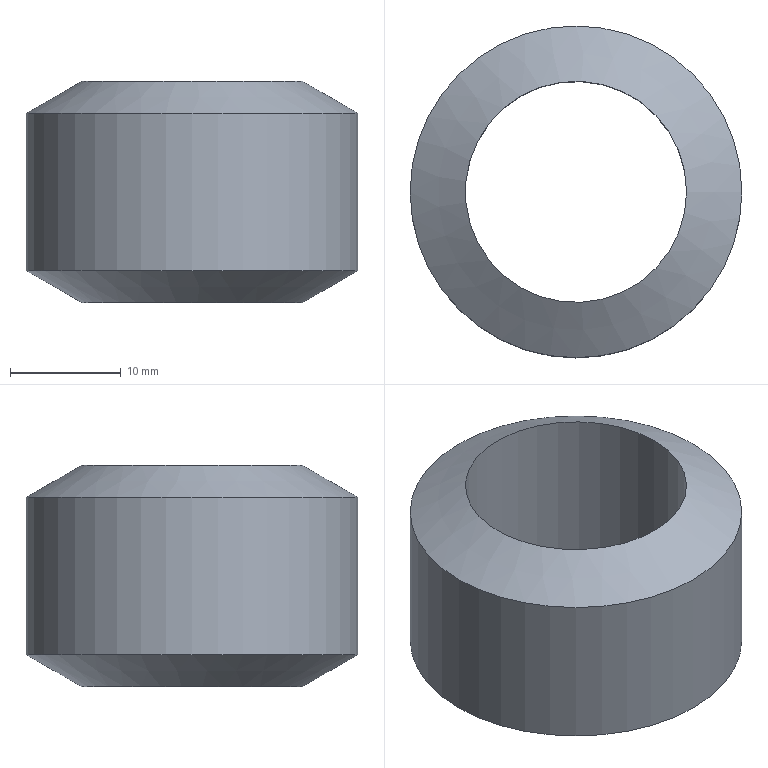Component | NX | PACKING | 1 solid | 4 faces | volume 6645 mm3 | cylinder 2 | cone 2 | commonest cylinder face diameters 30 x1 20 x1